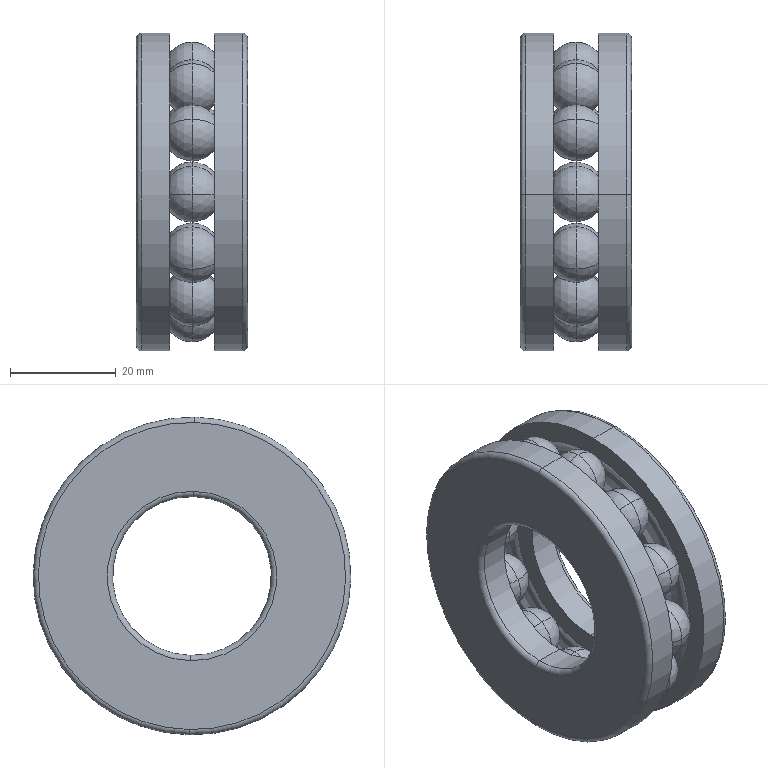Component | SolidWorks | 216InnerTubeAssembly-1_GB_T301-1995[ThrustBallBearing[51000]51306]-1 | 1 solid | 94 faces | volume 32155 mm3 | sphere 48 | torus 32 | cylinder 8 | plane 6 | commonest cylinder face diameters 60 x4 30 x2 32 x2